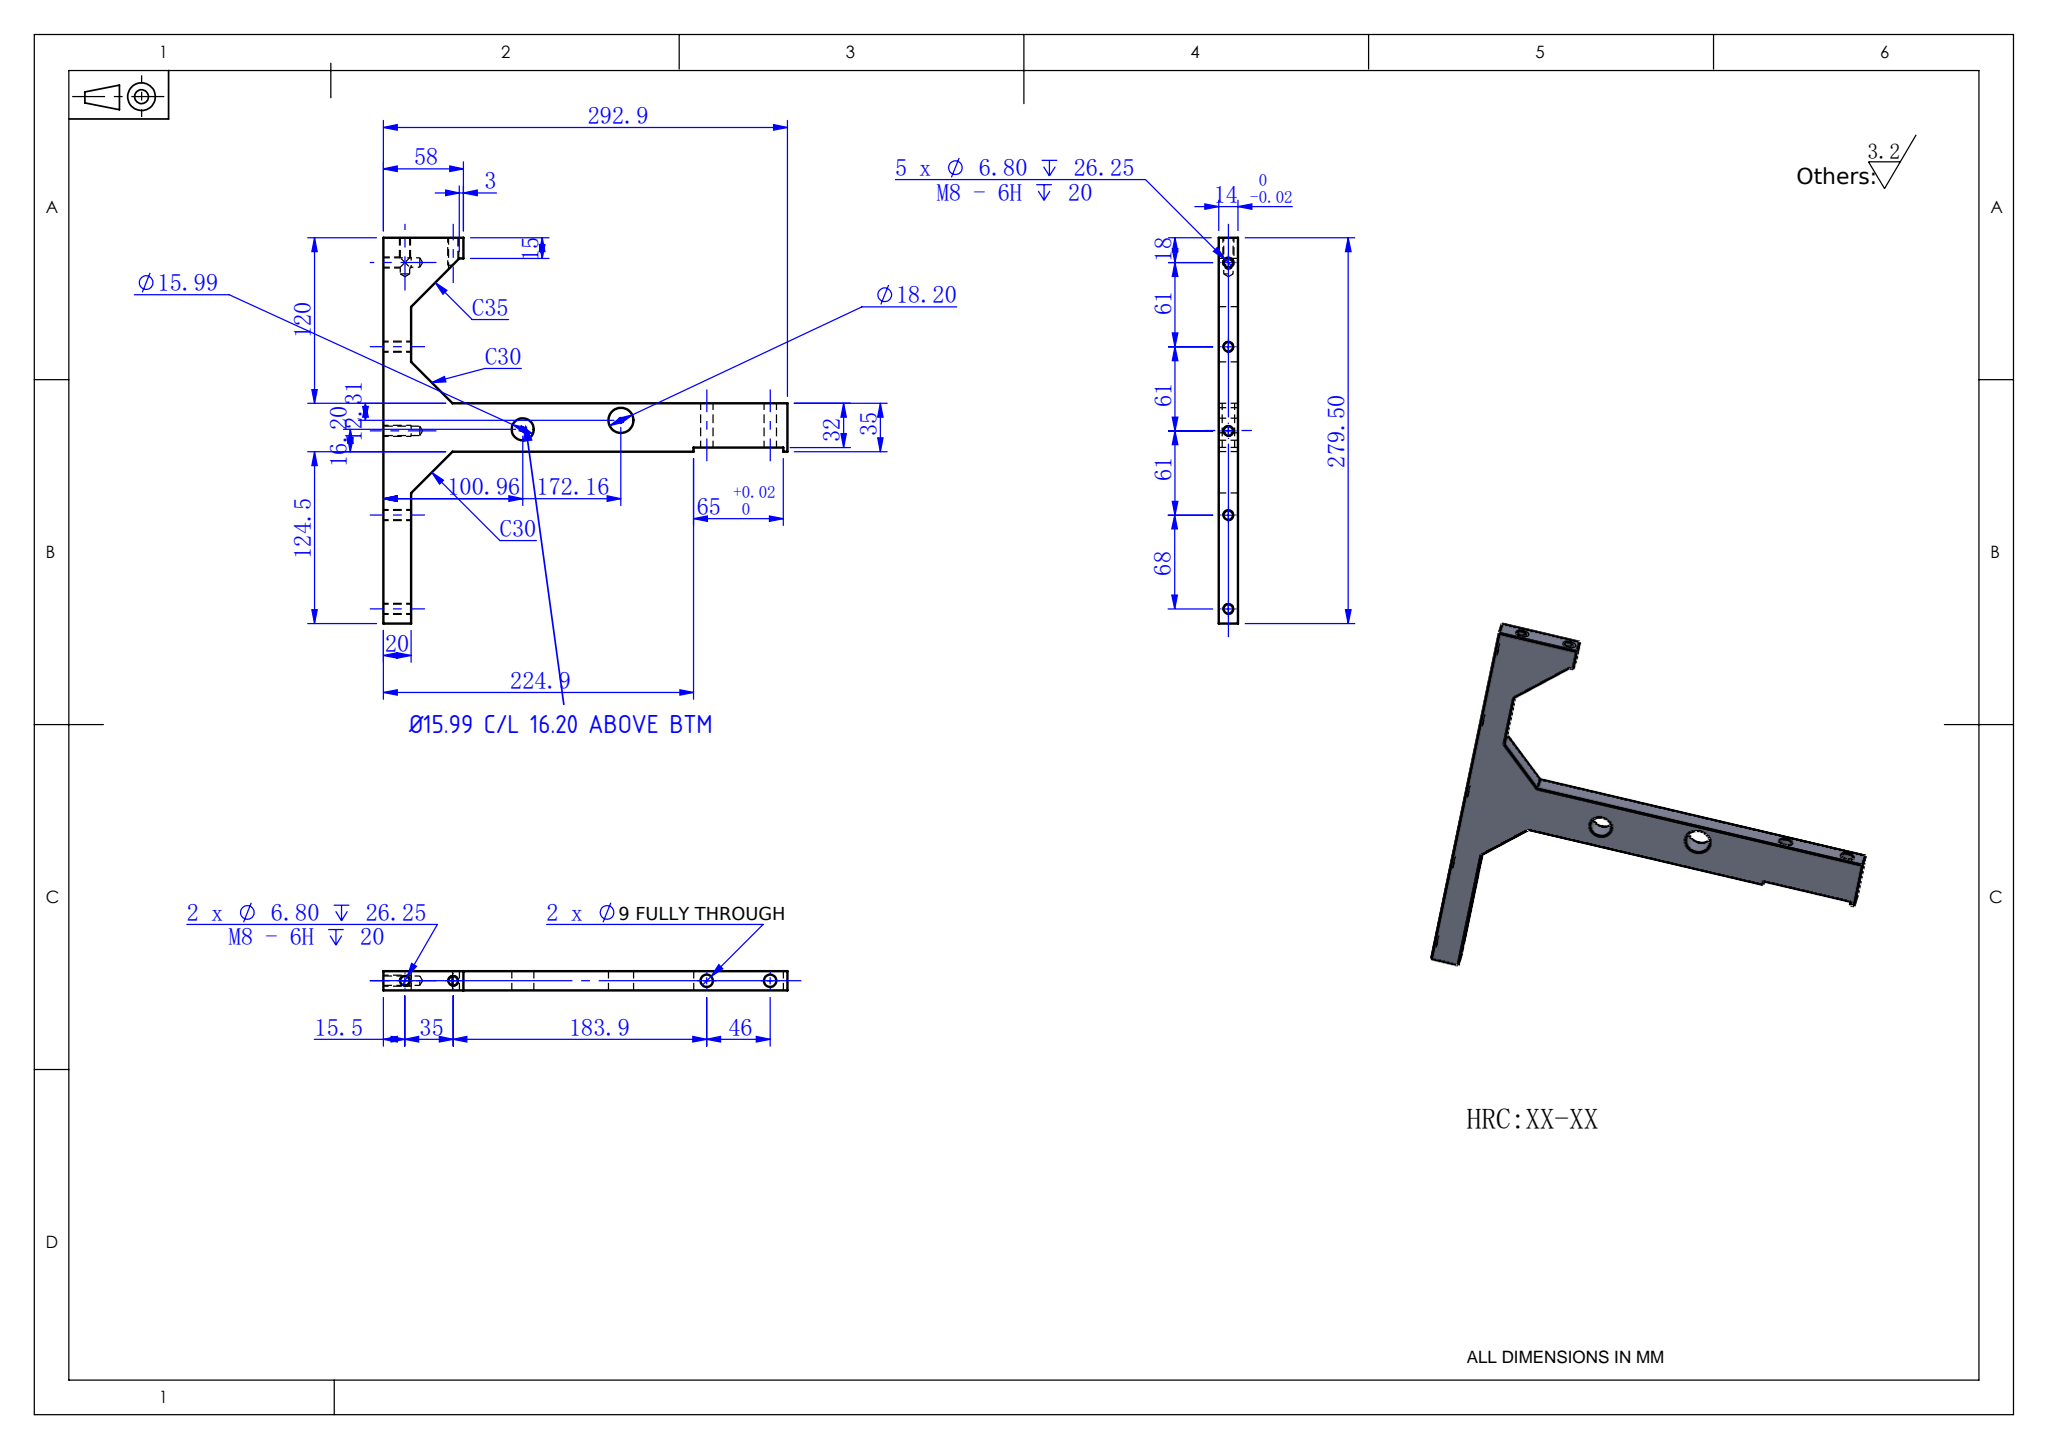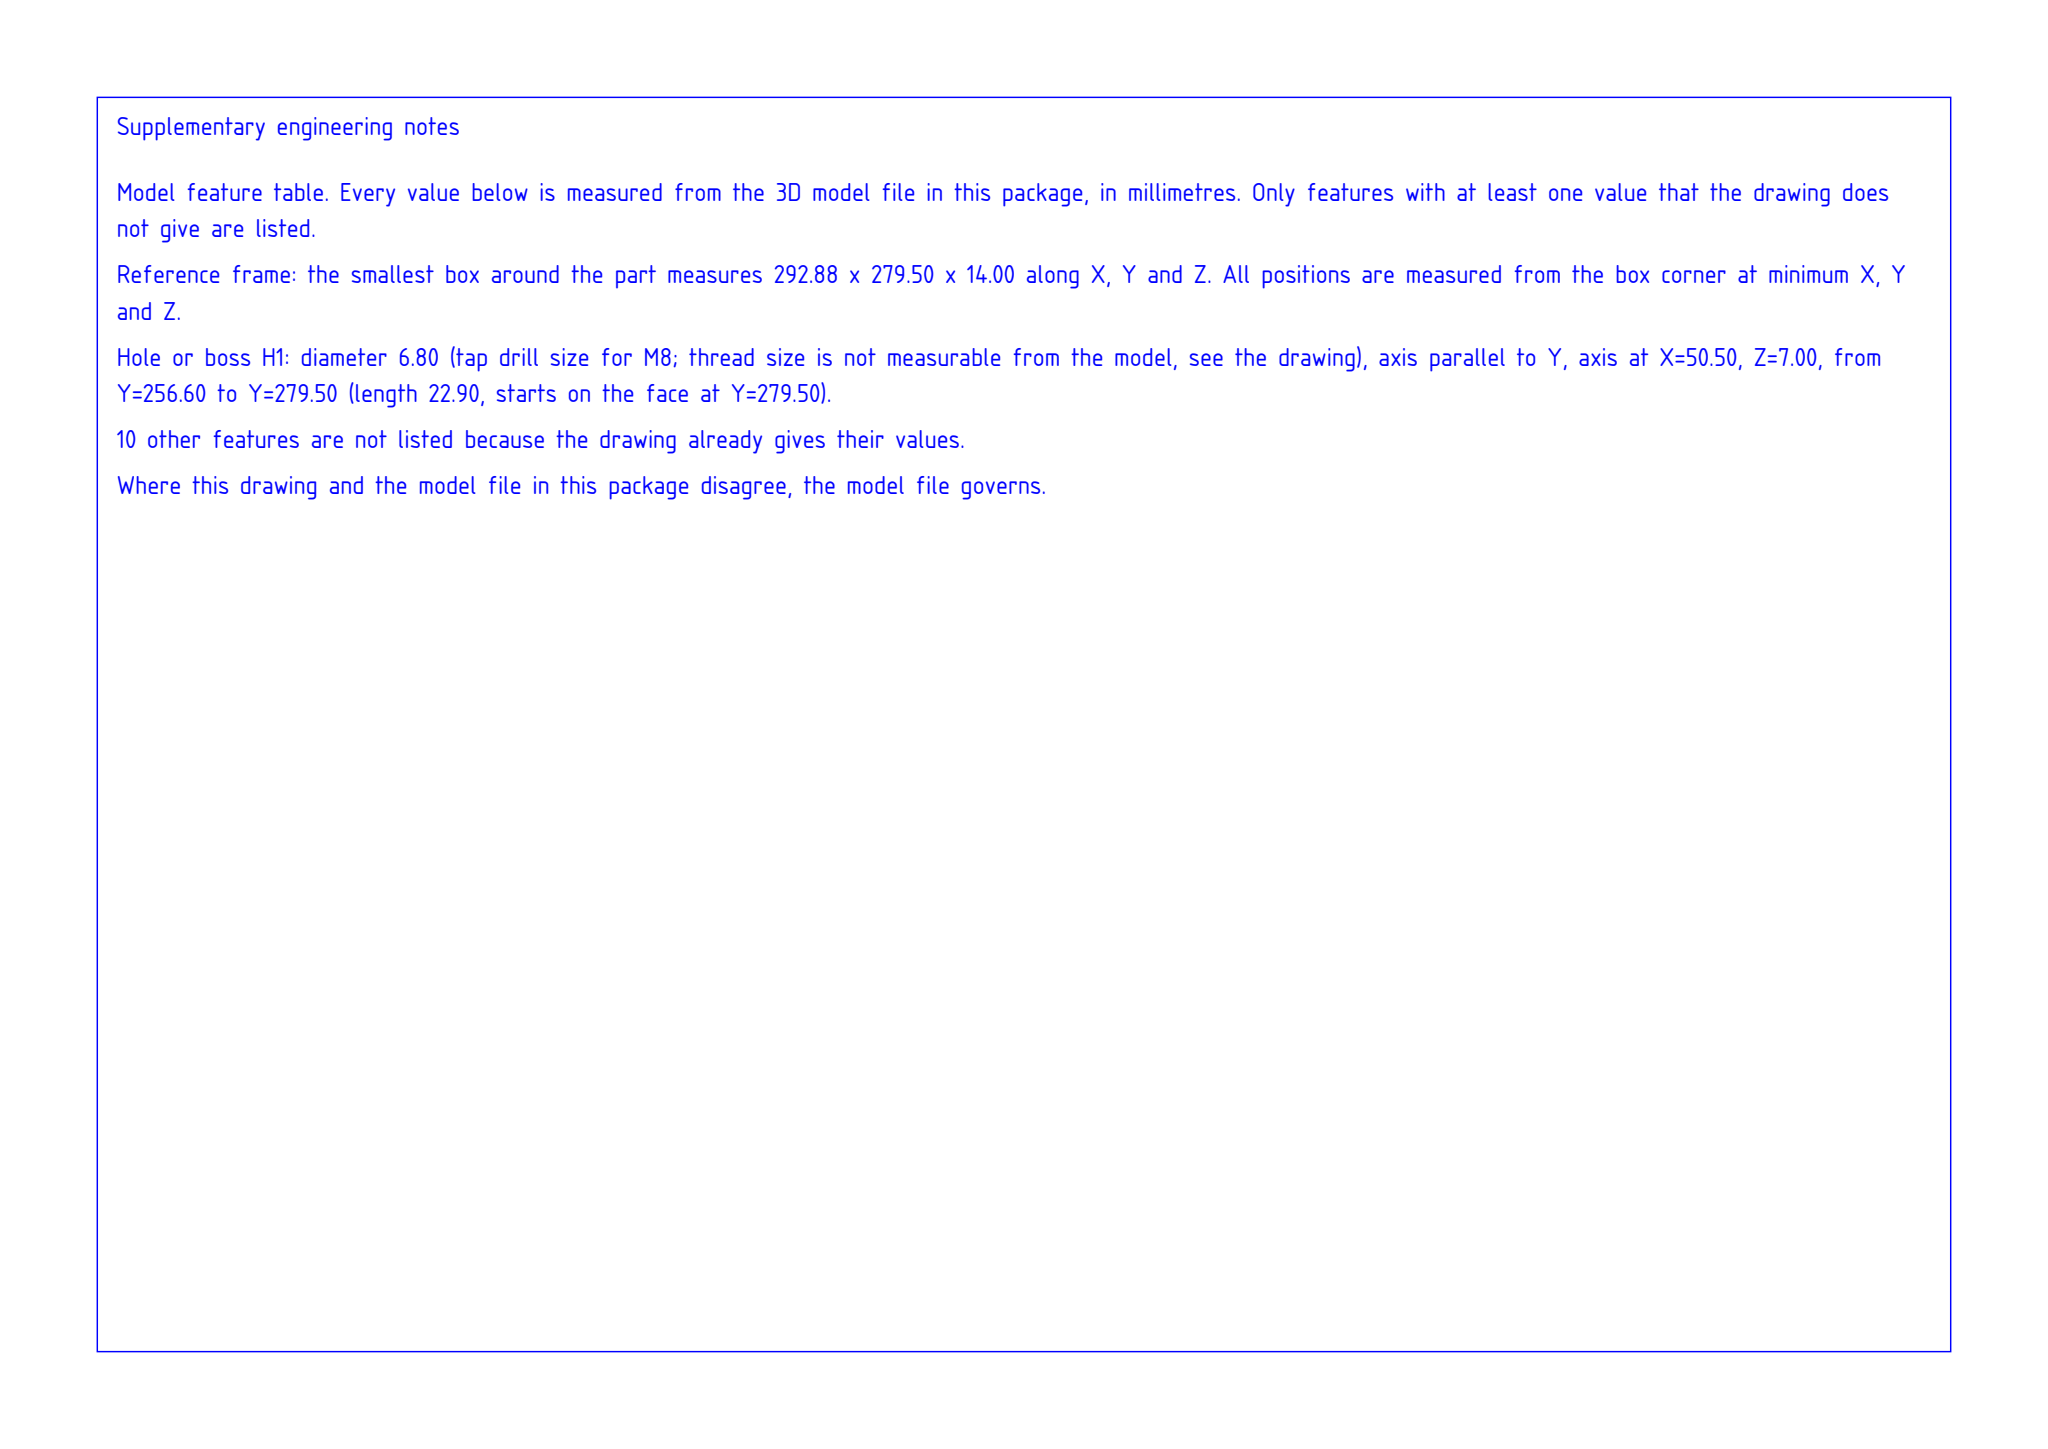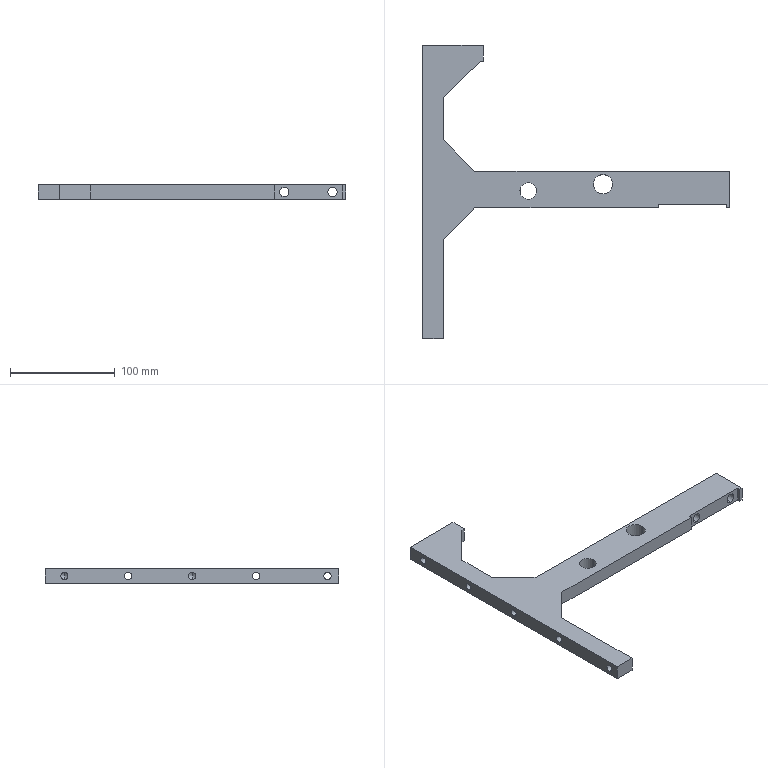Part | SolidWorks | mm | 1 solid | 51 faces | box 292.88 x 279.5 x 14 mm | volume 222260 mm3 | cylinder 26 | plane 19 | cone 6 | commonest cylinder face diameters 6.8 x18 9 x4 18.201 x2 15.989 x2
Drawing notes:
Ø15.99 C/L 16.20 ABOVE ARM BTM; Ø18.20 C/L 12.31 BELOW ARM TOP | from the solid: Ø15.989 axis y=140.7 vs arm btm face y=124.5 -> 16.20; Ø18.201 axis y=147.19 vs arm top face y=159.5 -> 12.31
build123d program:
from build123d import *

# Parameters (mm, degrees)
BOSS_EXTRUDE1_DEPTH      = 14
SKETCH2_W                = 14
SKETCH2_H                = 15
BOSS_EXTRUDE2_DEPTH      = 38
CHAMFER2_SIZE            = 35
M8_TAPPED_HOLE1_D        = 6.8
M8_TAPPED_HOLE1_DEPTH    = 26.25
M8_TAPPED_HOLE1_TIP      = 2.043
M8_TAPPED_HOLE2_D        = 6.8
M8_TAPPED_HOLE2_DEPTH    = 26.25
M8_TAPPED_HOLE2_TIP      = 2.043
CHAMFER3_SIZE            = 30
SKETCH7_W                = 65
SKETCH7_H                = 3
CUT_EXTRUDE1_DEPTH       = 619.732
F_9_0_9_DIAMETER_HOLE1_D = 9
SKETCH10_R               = 9.1
SKETCH10_R_2             = 7.994
CUT_EXTRUDE2_DEPTH       = 50


with BuildPart() as part:
    # Sketch1 → Boss-Extrude1 (new body)
    with BuildSketch(Plane.XY):
        Polygon((316.997, 93.278), (316.997, -26.722), (589.877, -26.722), (589.877, -61.722), (316.997, -61.722), (316.997, -186.222), (296.997, -186.222), (296.997, 93.278), align=None)
    extrude(amount=BOSS_EXTRUDE1_DEPTH)

    # Sketch2 → Boss-Extrude2 (add)
    with BuildSketch(Plane(origin=(316.997, 0, 0), x_dir=(0, 0, -1), z_dir=(1, 0, 0))):
        with Locations((-7, 85.778)):
            Rectangle(SKETCH2_W, SKETCH2_H)
    extrude(amount=BOSS_EXTRUDE2_DEPTH)

    # Chamfer2
    chamfer2_edges = [part.edges().sort_by_distance(p)[0] for p in [
        (316.997, 78.278, 7),
    ]]
    chamfer(chamfer2_edges, length=CHAMFER2_SIZE)

    # M8 Tapped Hole1
    with Locations(Plane(origin=(0, 93.278, 0), x_dir=(1, 0, 0), z_dir=(0, 1, 0))):
        with Locations((312.497, -7), (347.497, -7)):
            Hole(M8_TAPPED_HOLE1_D / 2, depth=M8_TAPPED_HOLE1_DEPTH)
            with Locations((0, 0, -(M8_TAPPED_HOLE1_DEPTH + M8_TAPPED_HOLE1_TIP / 2))):  # 118° drill point
                Cone(0, M8_TAPPED_HOLE1_D / 2, M8_TAPPED_HOLE1_TIP, mode=Mode.SUBTRACT)

    # M8 Tapped Hole2
    with Locations(Plane.ZY.offset(-296.997)):
        with Locations((7, 75.278), (7, 14.278), (7, -46.722), (7, -107.722), (7, -175.722)):
            Hole(M8_TAPPED_HOLE2_D / 2, depth=M8_TAPPED_HOLE2_DEPTH)
            with Locations((0, 0, -(M8_TAPPED_HOLE2_DEPTH + M8_TAPPED_HOLE2_TIP / 2))):  # 118° drill point
                Cone(0, M8_TAPPED_HOLE2_D / 2, M8_TAPPED_HOLE2_TIP, mode=Mode.SUBTRACT)

    # Chamfer3
    chamfer3_edges = [part.edges().sort_by_distance(p)[0] for p in [
        (316.997, -26.722, 7),
        (316.997, -61.722, 7),
    ]]
    chamfer(chamfer3_edges, length=CHAMFER3_SIZE)

    # Sketch7 → Cut-Extrude1 (cut, through all)
    with BuildSketch(Plane.XY.offset(14)):
        with Locations((554.377, -60.222)):
            Rectangle(SKETCH7_W, SKETCH7_H)
    extrude(amount=-CUT_EXTRUDE1_DEPTH, mode=Mode.SUBTRACT)

    # 9.0 _9_ Diameter Hole1 (through all)
    with Locations(Plane(origin=(0, -26.722, 0), x_dir=(1, 0, 0), z_dir=(0, 1, 0))):
        with Locations((577.377, -7), (531.377, -7)):
            Hole(F_9_0_9_DIAMETER_HOLE1_D / 2)

    # Sketch10 → Cut-Extrude2 (cut)
    with BuildSketch(Plane(origin=(0, 0, 0), x_dir=(-1, 0, 0), z_dir=(0, 0, -1))):
        with Locations((-469.155, -39.027)):
            Circle(SKETCH10_R)
        with Locations((-397.955, -45.524)):
            Circle(SKETCH10_R_2)
    extrude(amount=-CUT_EXTRUDE2_DEPTH, mode=Mode.SUBTRACT)


solid = part.part